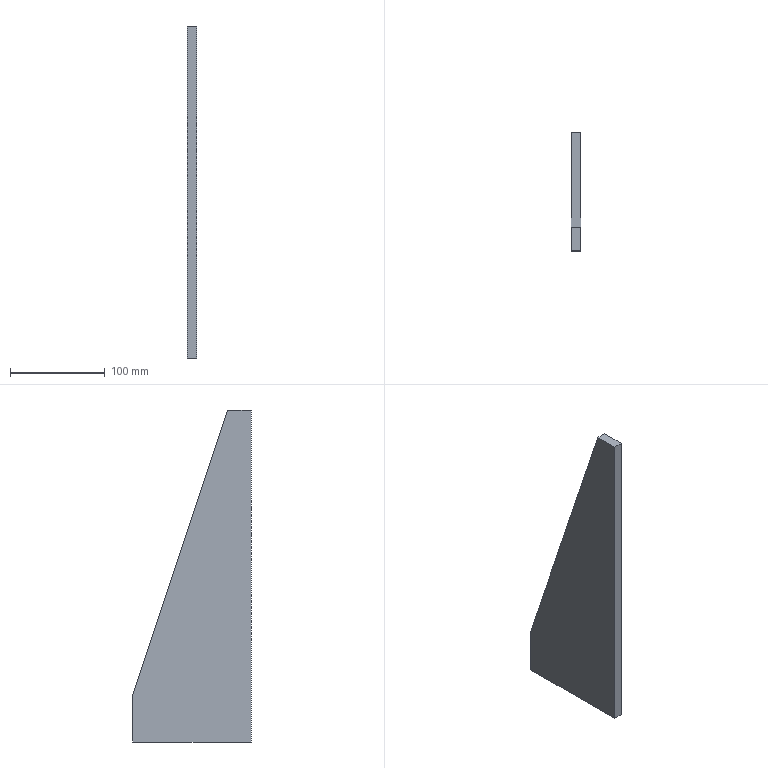Component | SolidWorks | Main-1_350X125X10-2 | 1 solid | 7 faces | box 10 x 125 x 350 mm | volume 287500 mm3 | plane 7 | material Plain Carbon Steel
STEP:
#1=COLOUR_RGB('',0.7922,0.8196,0.9333);
#2=FILL_AREA_STYLE_COLOUR('',#1);
#3=FILL_AREA_STYLE('',(#2));
#4=SURFACE_STYLE_FILL_AREA(#3);
#5=SURFACE_SIDE_STYLE('',(#4));
#6=SURFACE_STYLE_USAGE(.BOTH.,#5);
#7=PRESENTATION_STYLE_ASSIGNMENT((#6));
#8=CARTESIAN_POINT('',(-122.724,83.517,219.133));
#9=VERTEX_POINT('',#8);
#10=CARTESIAN_POINT('',(-122.724,83.517,205.353));
#11=VERTEX_POINT('',#10);
#12=CARTESIAN_POINT('',(-122.724,83.517,205.353));
#13=DIRECTION('',(-0.,0.,-1.));
#14=VECTOR('',#13,39.37);
#15=LINE('',#12,#14);
#16=EDGE_CURVE('',#9,#11,#15,.T.);
#17=ORIENTED_EDGE('',*,*,#16,.F.);
#18=CARTESIAN_POINT('',(-123.118,83.517,219.133));
#19=VERTEX_POINT('',#18);
#20=CARTESIAN_POINT('',(-123.118,83.517,219.133));
#21=DIRECTION('',(1.,0.,-0.));
#22=VECTOR('',#21,39.37);
#23=LINE('',#20,#22);
#24=EDGE_CURVE('',#19,#9,#23,.T.);
#25=ORIENTED_EDGE('',*,*,#24,.F.);
#26=CARTESIAN_POINT('',(-123.118,83.517,205.353));
#27=VERTEX_POINT('',#26);
#28=CARTESIAN_POINT('',(-123.118,83.517,205.353));
#29=DIRECTION('',(-0.,0.,-1.));
#30=VECTOR('',#29,39.37);
#31=LINE('',#28,#30);
#32=EDGE_CURVE('',#19,#27,#31,.T.);
#33=ORIENTED_EDGE('',*,*,#32,.T.);
#34=CARTESIAN_POINT('',(-123.118,83.517,205.353));
#35=DIRECTION('',(1.,0.,-0.));
#36=VECTOR('',#35,39.37);
#37=LINE('',#34,#36);
#38=EDGE_CURVE('',#27,#11,#37,.T.);
#39=ORIENTED_EDGE('',*,*,#38,.T.);
#40=EDGE_LOOP('',(#17,#25,#33,#39));
#41=FACE_OUTER_BOUND('',#40,.T.);
#42=CARTESIAN_POINT('',(-123.118,83.517,205.353));
#43=DIRECTION('',(0.,-1.,-0.));
#44=DIRECTION('',(-0.,0.,-1.));
#45=AXIS2_PLACEMENT_3D('',#42,#43,#44);
#46=PLANE('',#45);
#47=ADVANCED_FACE('',(#41),#46,.T.);
#48=CARTESIAN_POINT('',(-122.724,84.501,219.133));
#49=VERTEX_POINT('',#48);
#50=CARTESIAN_POINT('',(-122.724,83.517,219.133));
#51=DIRECTION('',(0.,-1.,-0.));
#52=VECTOR('',#51,39.37);
#53=LINE('',#50,#52);
#54=EDGE_CURVE('',#49,#9,#53,.T.);
#55=ORIENTED_EDGE('',*,*,#54,.F.);
#56=CARTESIAN_POINT('',(-123.118,84.501,219.133));
#57=VERTEX_POINT('',#56);
#58=CARTESIAN_POINT('',(-123.118,84.501,219.133));
#59=DIRECTION('',(1.,0.,-0.));
#60=VECTOR('',#59,39.37);
#61=LINE('',#58,#60);
#62=EDGE_CURVE('',#57,#49,#61,.T.);
#63=ORIENTED_EDGE('',*,*,#62,.F.);
#64=CARTESIAN_POINT('',(-123.118,83.517,219.133));
#65=DIRECTION('',(0.,-1.,-0.));
#66=VECTOR('',#65,39.37);
#67=LINE('',#64,#66);
#68=EDGE_CURVE('',#57,#19,#67,.T.);
#69=ORIENTED_EDGE('',*,*,#68,.T.);
#70=ORIENTED_EDGE('',*,*,#24,.T.);
#71=EDGE_LOOP('',(#55,#63,#69,#70));
#72=FACE_OUTER_BOUND('',#71,.T.);
#73=CARTESIAN_POINT('',(-123.118,83.517,219.133));
#74=DIRECTION('',(0.,-0.,1.));
#75=DIRECTION('',(0.,-1.,-0.));
#76=AXIS2_PLACEMENT_3D('',#73,#74,#75);
#77=PLANE('',#76);
#78=ADVANCED_FACE('',(#72),#77,.T.);
#79=CARTESIAN_POINT('',(-122.724,88.438,207.322));
#80=VERTEX_POINT('',#79);
#81=CARTESIAN_POINT('',(-122.724,84.501,219.133));
#82=DIRECTION('',(0.,-0.3162,0.9487));
#83=VECTOR('',#82,39.37);
#84=LINE('',#81,#83);
#85=EDGE_CURVE('',#80,#49,#84,.T.);
#86=ORIENTED_EDGE('',*,*,#85,.F.);
#87=CARTESIAN_POINT('',(-123.118,88.438,207.322));
#88=VERTEX_POINT('',#87);
#89=CARTESIAN_POINT('',(-123.118,88.438,207.322));
#90=DIRECTION('',(1.,0.,-0.));
#91=VECTOR('',#90,39.37);
#92=LINE('',#89,#91);
#93=EDGE_CURVE('',#88,#80,#92,.T.);
#94=ORIENTED_EDGE('',*,*,#93,.F.);
#95=CARTESIAN_POINT('',(-123.118,84.501,219.133));
#96=DIRECTION('',(0.,-0.3162,0.9487));
#97=VECTOR('',#96,39.37);
#98=LINE('',#95,#97);
#99=EDGE_CURVE('',#88,#57,#98,.T.);
#100=ORIENTED_EDGE('',*,*,#99,.T.);
#101=ORIENTED_EDGE('',*,*,#62,.T.);
#102=EDGE_LOOP('',(#86,#94,#100,#101));
#103=FACE_OUTER_BOUND('',#102,.T.);
#104=CARTESIAN_POINT('',(-123.118,84.501,219.133));
#105=DIRECTION('',(-0.,0.9487,0.3162));
#106=DIRECTION('',(0.,-0.3162,0.9487));
#107=AXIS2_PLACEMENT_3D('',#104,#105,#106);
#108=PLANE('',#107);
#109=ADVANCED_FACE('',(#103),#108,.T.);
#110=CARTESIAN_POINT('',(-122.724,88.438,205.353));
#111=VERTEX_POINT('',#110);
#112=CARTESIAN_POINT('',(-122.724,88.438,207.322));
#113=DIRECTION('',(0.,-0.,1.));
#114=VECTOR('',#113,39.37);
#115=LINE('',#112,#114);
#116=EDGE_CURVE('',#111,#80,#115,.T.);
#117=ORIENTED_EDGE('',*,*,#116,.F.);
#118=CARTESIAN_POINT('',(-123.118,88.438,205.353));
#119=VERTEX_POINT('',#118);
#120=CARTESIAN_POINT('',(-123.118,88.438,205.353));
#121=DIRECTION('',(1.,0.,-0.));
#122=VECTOR('',#121,39.37);
#123=LINE('',#120,#122);
#124=EDGE_CURVE('',#119,#111,#123,.T.);
#125=ORIENTED_EDGE('',*,*,#124,.F.);
#126=CARTESIAN_POINT('',(-123.118,88.438,207.322));
#127=DIRECTION('',(0.,-0.,1.));
#128=VECTOR('',#127,39.37);
#129=LINE('',#126,#128);
#130=EDGE_CURVE('',#119,#88,#129,.T.);
#131=ORIENTED_EDGE('',*,*,#130,.T.);
#132=ORIENTED_EDGE('',*,*,#93,.T.);
#133=EDGE_LOOP('',(#117,#125,#131,#132));
#134=FACE_OUTER_BOUND('',#133,.T.);
#135=CARTESIAN_POINT('',(-123.118,88.438,207.322));
#136=DIRECTION('',(-0.,1.,0.));
#137=DIRECTION('',(0.,-0.,1.));
#138=AXIS2_PLACEMENT_3D('',#135,#136,#137);
#139=PLANE('',#138);
#140=ADVANCED_FACE('',(#134),#139,.T.);
#141=CARTESIAN_POINT('',(-122.724,88.438,205.353));
#142=DIRECTION('',(-0.,1.,0.));
#143=VECTOR('',#142,39.37);
#144=LINE('',#141,#143);
#145=EDGE_CURVE('',#11,#111,#144,.T.);
#146=ORIENTED_EDGE('',*,*,#145,.F.);
#147=ORIENTED_EDGE('',*,*,#38,.F.);
#148=CARTESIAN_POINT('',(-123.118,88.438,205.353));
#149=DIRECTION('',(-0.,1.,0.));
#150=VECTOR('',#149,39.37);
#151=LINE('',#148,#150);
#152=EDGE_CURVE('',#27,#119,#151,.T.);
#153=ORIENTED_EDGE('',*,*,#152,.T.);
#154=ORIENTED_EDGE('',*,*,#124,.T.);
#155=EDGE_LOOP('',(#146,#147,#153,#154));
#156=FACE_OUTER_BOUND('',#155,.T.);
#157=CARTESIAN_POINT('',(-123.118,88.438,205.353));
#158=DIRECTION('',(-0.,0.,-1.));
#159=DIRECTION('',(-0.,1.,0.));
#160=AXIS2_PLACEMENT_3D('',#157,#158,#159);
#161=PLANE('',#160);
#162=ADVANCED_FACE('',(#156),#161,.T.);
#163=ORIENTED_EDGE('',*,*,#32,.F.);
#164=ORIENTED_EDGE('',*,*,#68,.F.);
#165=ORIENTED_EDGE('',*,*,#99,.F.);
#166=ORIENTED_EDGE('',*,*,#130,.F.);
#167=ORIENTED_EDGE('',*,*,#152,.F.);
#168=EDGE_LOOP('',(#163,#164,#165,#166,#167));
#169=FACE_OUTER_BOUND('',#168,.T.);
#170=CARTESIAN_POINT('',(-123.118,83.517,219.133));
#171=DIRECTION('',(-1.,-0.,0.));
#172=DIRECTION('',(0.,-0.,1.));
#173=AXIS2_PLACEMENT_3D('',#170,#171,#172);
#174=PLANE('',#173);
#175=ADVANCED_FACE('',(#169),#174,.T.);
#176=ORIENTED_EDGE('',*,*,#16,.T.);
#177=ORIENTED_EDGE('',*,*,#145,.T.);
#178=ORIENTED_EDGE('',*,*,#116,.T.);
#179=ORIENTED_EDGE('',*,*,#85,.T.);
#180=ORIENTED_EDGE('',*,*,#54,.T.);
#181=EDGE_LOOP('',(#176,#177,#178,#179,#180));
#182=FACE_OUTER_BOUND('',#181,.T.);
#183=CARTESIAN_POINT('',(-122.724,83.517,219.133));
#184=DIRECTION('',(-1.,-0.,0.));
#185=DIRECTION('',(0.,-0.,1.));
#186=AXIS2_PLACEMENT_3D('',#183,#184,#185);
#187=PLANE('',#186);
#188=ADVANCED_FACE('',(#182),#187,.F.);
#189=CLOSED_SHELL('',(#47,#78,#109,#140,#162,#175,#188));
#190=MANIFOLD_SOLID_BREP('',#189);
#191=STYLED_ITEM('',(#7),#190);
#192=PRESENTATION_LAYER_ASSIGNMENT('','',(#191));
#193=(LENGTH_UNIT()NAMED_UNIT(*)SI_UNIT($,.METRE.));
#194=LENGTH_MEASURE_WITH_UNIT(LENGTH_MEASURE(0.0254),#193);
#195=DIMENSIONAL_EXPONENTS(1.,0.,0.,0.,0.,0.,0.);
#196=(CONVERSION_BASED_UNIT('',#194)LENGTH_UNIT()NAMED_UNIT(#195));
#197=UNCERTAINTY_MEASURE_WITH_UNIT(LENGTH_MEASURE(0.00001),#196,'','');
#198=(NAMED_UNIT(*)PLANE_ANGLE_UNIT()SI_UNIT($,.RADIAN.));
#199=(NAMED_UNIT(*)SI_UNIT($,.STERADIAN.)SOLID_ANGLE_UNIT());
#200=(GEOMETRIC_REPRESENTATION_CONTEXT(3)GLOBAL_UNCERTAINTY_ASSIGNED_CONTEXT((#197))GLOBAL_UNIT_ASSIGNED_CONTEXT((#196,#198,#199))REPRESENTATION_CONTEXT('',''));
#201=MECHANICAL_DESIGN_GEOMETRIC_PRESENTATION_REPRESENTATION('',(#191),#200);
#202=CARTESIAN_POINT('',(0.,0.,0.));
#203=DIRECTION('',(0.,0.,1.));
#204=DIRECTION('',(1.,0.,0.));
#205=AXIS2_PLACEMENT_3D('',#202,#203,#204);
#206=(LENGTH_UNIT()NAMED_UNIT(*)SI_UNIT($,.METRE.));
#207=LENGTH_MEASURE_WITH_UNIT(LENGTH_MEASURE(0.0254),#206);
#208=DIMENSIONAL_EXPONENTS(1.,0.,0.,0.,0.,0.,0.);
#209=(CONVERSION_BASED_UNIT('',#207)LENGTH_UNIT()NAMED_UNIT(#208));
#210=UNCERTAINTY_MEASURE_WITH_UNIT(LENGTH_MEASURE(0.00001),#209,'','');
#211=(NAMED_UNIT(*)PLANE_ANGLE_UNIT()SI_UNIT($,.RADIAN.));
#212=(NAMED_UNIT(*)SI_UNIT($,.STERADIAN.)SOLID_ANGLE_UNIT());
#213=(GEOMETRIC_REPRESENTATION_CONTEXT(3)GLOBAL_UNCERTAINTY_ASSIGNED_CONTEXT((#210))GLOBAL_UNIT_ASSIGNED_CONTEXT((#209,#211,#212))REPRESENTATION_CONTEXT('',''));
#214=ADVANCED_BREP_SHAPE_REPRESENTATION('',(#190,#205),#213);